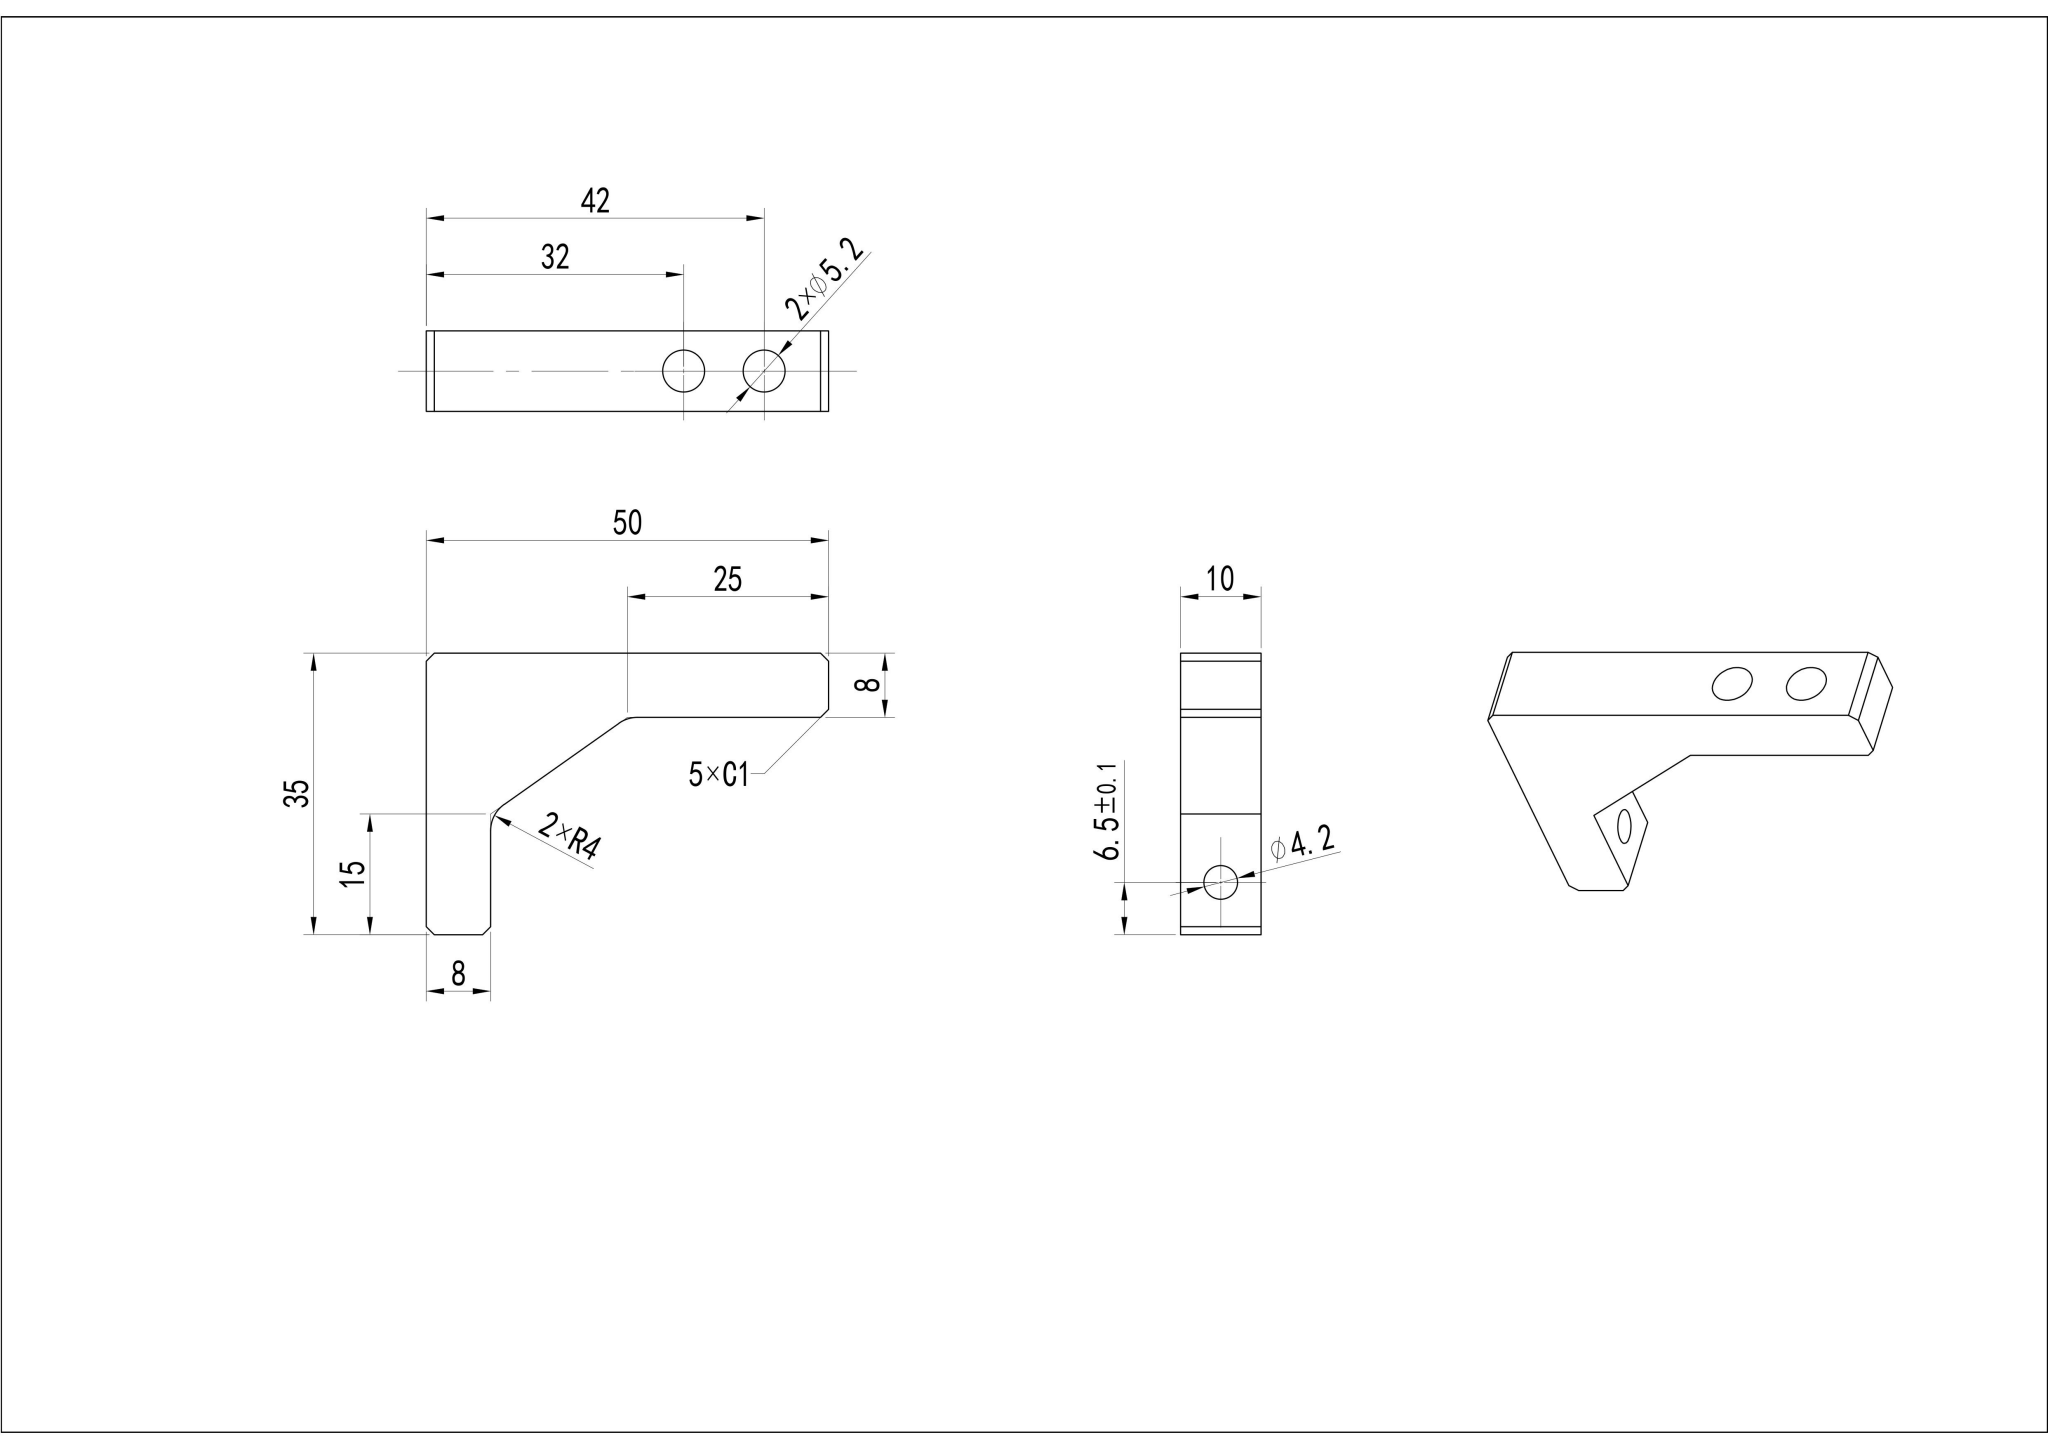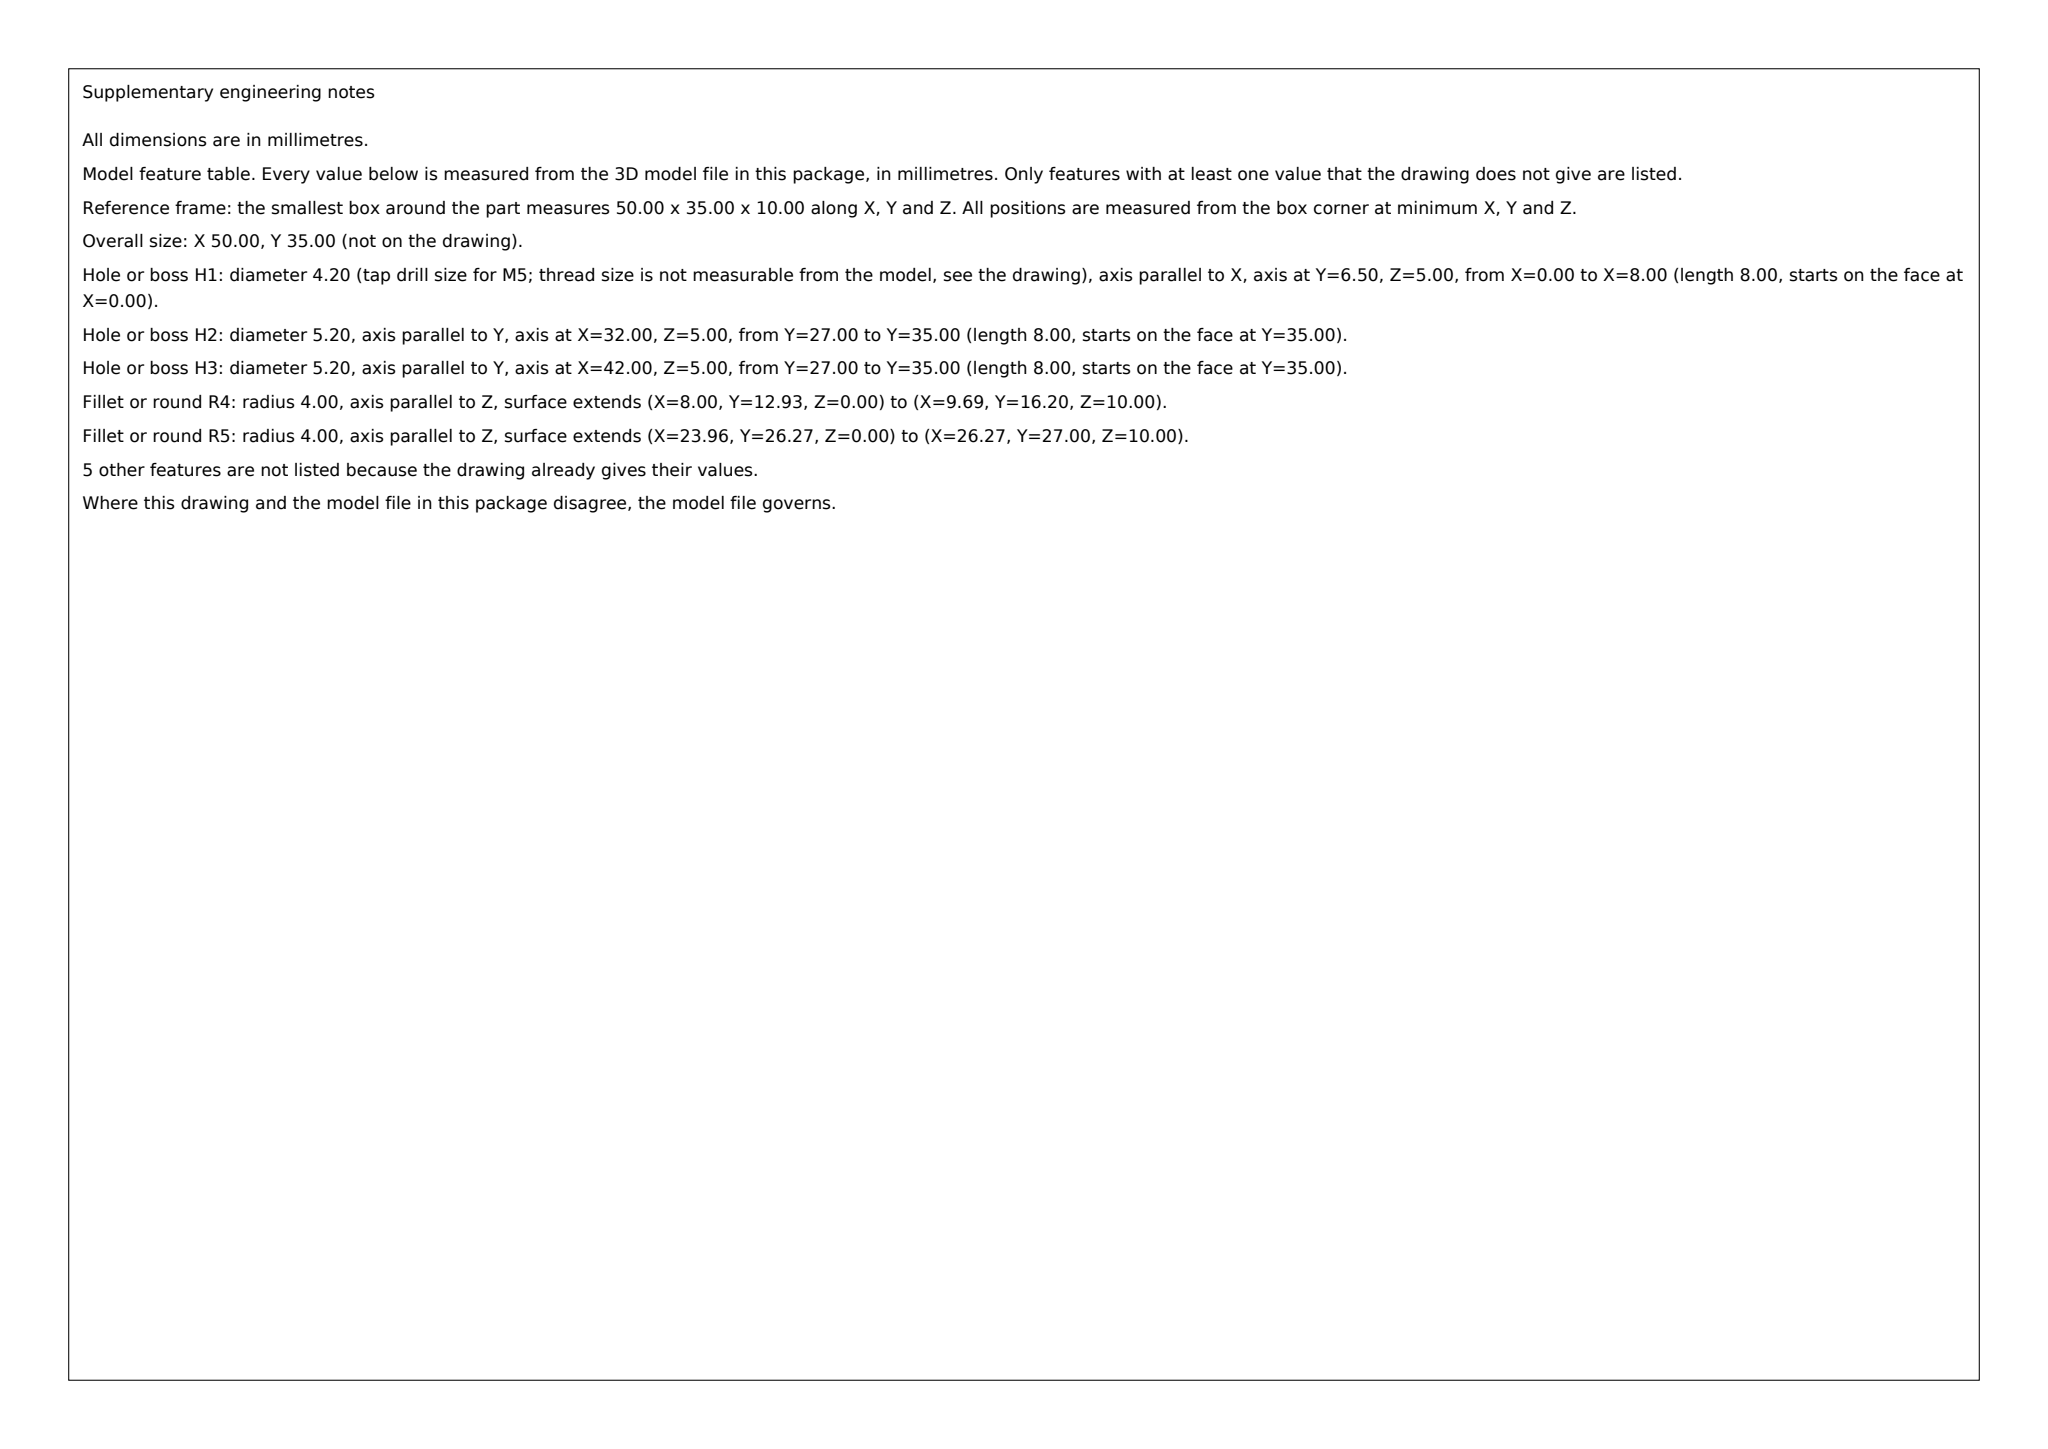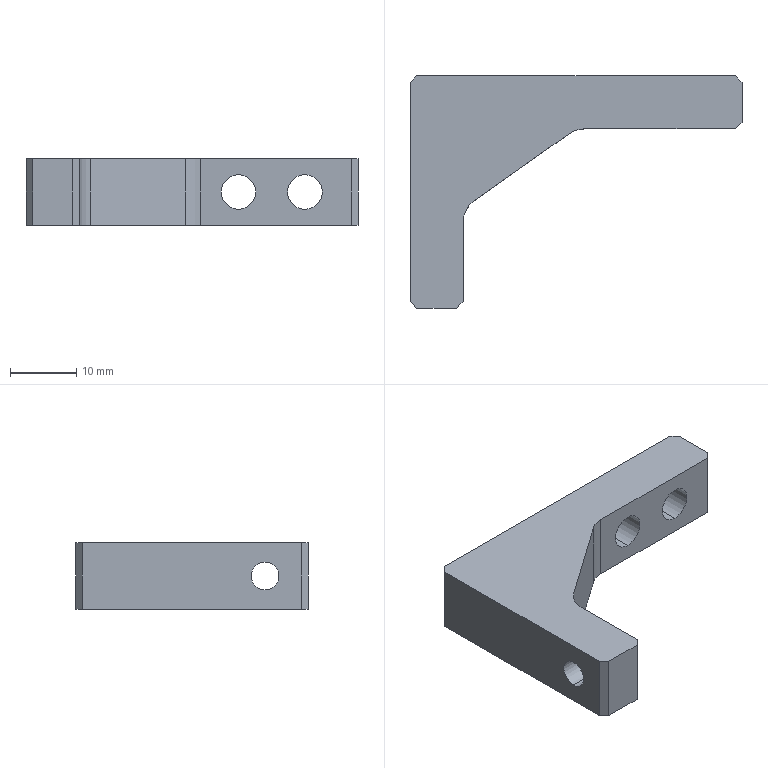Part | SolidWorks | mm | 1 solid | 22 faces | box 50 x 35 x 10 mm | volume 6712 mm3 | plane 14 | cylinder 8 | commonest cylinder face diameters 5.2 x4 4.2 x2 8 x2
STEP:
#1=CARTESIAN_POINT('',(-8.828,-14.732,2.1));
#2=VERTEX_POINT('',#1);
#3=CARTESIAN_POINT('',(-8.828,-14.732,-2.1));
#4=VERTEX_POINT('',#3);
#5=CARTESIAN_POINT('',(-8.828,-14.732,0.));
#6=DIRECTION('',(1.,0.,0.));
#7=DIRECTION('',(0.,0.,1.));
#8=AXIS2_PLACEMENT_3D('',#5,#6,#7);
#9=CIRCLE('',#8,2.1);
#10=EDGE_CURVE('',#2,#4,#9,.T.);
#11=ORIENTED_EDGE('',*,*,#10,.T.);
#12=CARTESIAN_POINT('',(-16.828,-14.732,-2.1));
#13=VERTEX_POINT('',#12);
#14=CARTESIAN_POINT('',(-6.828,-14.732,-2.1));
#15=DIRECTION('',(-1.,0.,0.));
#16=VECTOR('',#15,1000.);
#17=LINE('',#14,#16);
#18=EDGE_CURVE('',#4,#13,#17,.T.);
#19=ORIENTED_EDGE('',*,*,#18,.T.);
#20=CARTESIAN_POINT('',(-16.828,-14.732,2.1));
#21=VERTEX_POINT('',#20);
#22=CARTESIAN_POINT('',(-16.828,-14.732,0.));
#23=DIRECTION('',(-1.,0.,0.));
#24=DIRECTION('',(0.,0.,1.));
#25=AXIS2_PLACEMENT_3D('',#22,#23,#24);
#26=CIRCLE('',#25,2.1);
#27=EDGE_CURVE('',#13,#21,#26,.T.);
#28=ORIENTED_EDGE('',*,*,#27,.T.);
#29=CARTESIAN_POINT('',(-6.828,-14.732,2.1));
#30=DIRECTION('',(-1.,0.,0.));
#31=VECTOR('',#30,1000.);
#32=LINE('',#29,#31);
#33=EDGE_CURVE('',#2,#21,#32,.T.);
#34=ORIENTED_EDGE('',*,*,#33,.F.);
#35=EDGE_LOOP('',(#11,#19,#28,#34));
#36=FACE_OUTER_BOUND('',#35,.T.);
#37=CARTESIAN_POINT('',(-6.828,-14.732,0.));
#38=DIRECTION('',(-1.,0.,0.));
#39=DIRECTION('',(0.,0.,1.));
#40=AXIS2_PLACEMENT_3D('',#37,#38,#39);
#41=CYLINDRICAL_SURFACE('',#40,2.1);
#42=ADVANCED_FACE('',(#36),#41,.F.);
#43=CARTESIAN_POINT('',(15.172,5.768,2.6));
#44=VERTEX_POINT('',#43);
#45=CARTESIAN_POINT('',(15.172,5.768,-2.6));
#46=VERTEX_POINT('',#45);
#47=CARTESIAN_POINT('',(15.172,5.768,0.));
#48=DIRECTION('',(0.,-1.,0.));
#49=DIRECTION('',(0.,0.,1.));
#50=AXIS2_PLACEMENT_3D('',#47,#48,#49);
#51=CIRCLE('',#50,2.6);
#52=EDGE_CURVE('',#44,#46,#51,.T.);
#53=ORIENTED_EDGE('',*,*,#52,.T.);
#54=CARTESIAN_POINT('',(15.172,13.768,-2.6));
#55=VERTEX_POINT('',#54);
#56=CARTESIAN_POINT('',(15.172,3.768,-2.6));
#57=DIRECTION('',(0.,1.,0.));
#58=VECTOR('',#57,1000.);
#59=LINE('',#56,#58);
#60=EDGE_CURVE('',#46,#55,#59,.T.);
#61=ORIENTED_EDGE('',*,*,#60,.T.);
#62=CARTESIAN_POINT('',(15.172,13.768,2.6));
#63=VERTEX_POINT('',#62);
#64=CARTESIAN_POINT('',(15.172,13.768,0.));
#65=DIRECTION('',(0.,1.,0.));
#66=DIRECTION('',(0.,0.,1.));
#67=AXIS2_PLACEMENT_3D('',#64,#65,#66);
#68=CIRCLE('',#67,2.6);
#69=EDGE_CURVE('',#55,#63,#68,.T.);
#70=ORIENTED_EDGE('',*,*,#69,.T.);
#71=CARTESIAN_POINT('',(15.172,3.768,2.6));
#72=DIRECTION('',(0.,1.,0.));
#73=VECTOR('',#72,1000.);
#74=LINE('',#71,#73);
#75=EDGE_CURVE('',#44,#63,#74,.T.);
#76=ORIENTED_EDGE('',*,*,#75,.F.);
#77=EDGE_LOOP('',(#53,#61,#70,#76));
#78=FACE_OUTER_BOUND('',#77,.T.);
#79=CARTESIAN_POINT('',(15.172,3.768,0.));
#80=DIRECTION('',(0.,1.,0.));
#81=DIRECTION('',(0.,0.,1.));
#82=AXIS2_PLACEMENT_3D('',#79,#80,#81);
#83=CYLINDRICAL_SURFACE('',#82,2.6);
#84=ADVANCED_FACE('',(#78),#83,.F.);
#85=CARTESIAN_POINT('',(25.172,5.768,2.6));
#86=VERTEX_POINT('',#85);
#87=CARTESIAN_POINT('',(25.172,5.768,-2.6));
#88=VERTEX_POINT('',#87);
#89=CARTESIAN_POINT('',(25.172,5.768,0.));
#90=DIRECTION('',(0.,-1.,0.));
#91=DIRECTION('',(0.,0.,1.));
#92=AXIS2_PLACEMENT_3D('',#89,#90,#91);
#93=CIRCLE('',#92,2.6);
#94=EDGE_CURVE('',#86,#88,#93,.T.);
#95=ORIENTED_EDGE('',*,*,#94,.T.);
#96=CARTESIAN_POINT('',(25.172,13.768,-2.6));
#97=VERTEX_POINT('',#96);
#98=CARTESIAN_POINT('',(25.172,3.768,-2.6));
#99=DIRECTION('',(0.,1.,0.));
#100=VECTOR('',#99,1000.);
#101=LINE('',#98,#100);
#102=EDGE_CURVE('',#88,#97,#101,.T.);
#103=ORIENTED_EDGE('',*,*,#102,.T.);
#104=CARTESIAN_POINT('',(25.172,13.768,2.6));
#105=VERTEX_POINT('',#104);
#106=CARTESIAN_POINT('',(25.172,13.768,0.));
#107=DIRECTION('',(0.,1.,0.));
#108=DIRECTION('',(0.,0.,1.));
#109=AXIS2_PLACEMENT_3D('',#106,#107,#108);
#110=CIRCLE('',#109,2.6);
#111=EDGE_CURVE('',#97,#105,#110,.T.);
#112=ORIENTED_EDGE('',*,*,#111,.T.);
#113=CARTESIAN_POINT('',(25.172,3.768,2.6));
#114=DIRECTION('',(0.,1.,0.));
#115=VECTOR('',#114,1000.);
#116=LINE('',#113,#115);
#117=EDGE_CURVE('',#86,#105,#116,.T.);
#118=ORIENTED_EDGE('',*,*,#117,.F.);
#119=EDGE_LOOP('',(#95,#103,#112,#118));
#120=FACE_OUTER_BOUND('',#119,.T.);
#121=CARTESIAN_POINT('',(25.172,3.768,0.));
#122=DIRECTION('',(0.,1.,0.));
#123=DIRECTION('',(0.,0.,1.));
#124=AXIS2_PLACEMENT_3D('',#121,#122,#123);
#125=CYLINDRICAL_SURFACE('',#124,2.6);
#126=ADVANCED_FACE('',(#120),#125,.F.);
#127=CARTESIAN_POINT('',(-16.828,-20.232,5.));
#128=VERTEX_POINT('',#127);
#129=CARTESIAN_POINT('',(-15.828,-21.232,5.));
#130=VERTEX_POINT('',#129);
#131=CARTESIAN_POINT('',(-16.828,-20.232,5.));
#132=DIRECTION('',(0.7071,-0.7071,0.));
#133=VECTOR('',#132,1000.);
#134=LINE('',#131,#133);
#135=EDGE_CURVE('',#128,#130,#134,.T.);
#136=ORIENTED_EDGE('',*,*,#135,.T.);
#137=CARTESIAN_POINT('',(-9.828,-21.232,5.));
#138=VERTEX_POINT('',#137);
#139=CARTESIAN_POINT('',(-4.828,-21.232,5.));
#140=DIRECTION('',(-1.,0.,0.));
#141=VECTOR('',#140,1000.);
#142=LINE('',#139,#141);
#143=EDGE_CURVE('',#138,#130,#142,.T.);
#144=ORIENTED_EDGE('',*,*,#143,.F.);
#145=CARTESIAN_POINT('',(-8.828,-20.232,5.));
#146=VERTEX_POINT('',#145);
#147=CARTESIAN_POINT('',(-9.828,-21.232,5.));
#148=DIRECTION('',(0.7071,0.7071,0.));
#149=VECTOR('',#148,1000.);
#150=LINE('',#147,#149);
#151=EDGE_CURVE('',#138,#146,#150,.T.);
#152=ORIENTED_EDGE('',*,*,#151,.T.);
#153=CARTESIAN_POINT('',(-8.828,-8.304,5.));
#154=VERTEX_POINT('',#153);
#155=CARTESIAN_POINT('',(-8.828,-8.304,5.));
#156=DIRECTION('',(0.,-1.,0.));
#157=VECTOR('',#156,1000.);
#158=LINE('',#155,#157);
#159=EDGE_CURVE('',#154,#146,#158,.T.);
#160=ORIENTED_EDGE('',*,*,#159,.F.);
#161=CARTESIAN_POINT('',(-7.135,-5.036,5.));
#162=VERTEX_POINT('',#161);
#163=CARTESIAN_POINT('',(-4.828,-8.304,5.));
#164=DIRECTION('',(0.,0.,1.));
#165=DIRECTION('',(-1.,0.,0.));
#166=AXIS2_PLACEMENT_3D('',#163,#164,#165);
#167=CIRCLE('',#166,4.);
#168=EDGE_CURVE('',#162,#154,#167,.T.);
#169=ORIENTED_EDGE('',*,*,#168,.F.);
#170=CARTESIAN_POINT('',(7.135,5.036,5.));
#171=VERTEX_POINT('',#170);
#172=CARTESIAN_POINT('',(7.135,5.036,5.));
#173=DIRECTION('',(-0.817,-0.5767,0.));
#174=VECTOR('',#173,1000.);
#175=LINE('',#172,#174);
#176=EDGE_CURVE('',#171,#162,#175,.T.);
#177=ORIENTED_EDGE('',*,*,#176,.F.);
#178=CARTESIAN_POINT('',(9.442,5.768,5.));
#179=VERTEX_POINT('',#178);
#180=CARTESIAN_POINT('',(9.442,1.768,5.));
#181=DIRECTION('',(0.,0.,1.));
#182=DIRECTION('',(-1.,0.,0.));
#183=AXIS2_PLACEMENT_3D('',#180,#181,#182);
#184=CIRCLE('',#183,4.);
#185=EDGE_CURVE('',#179,#171,#184,.T.);
#186=ORIENTED_EDGE('',*,*,#185,.F.);
#187=CARTESIAN_POINT('',(32.172,5.768,5.));
#188=VERTEX_POINT('',#187);
#189=CARTESIAN_POINT('',(-4.828,5.768,5.));
#190=DIRECTION('',(-1.,0.,0.));
#191=VECTOR('',#190,1000.);
#192=LINE('',#189,#191);
#193=EDGE_CURVE('',#188,#179,#192,.T.);
#194=ORIENTED_EDGE('',*,*,#193,.F.);
#195=CARTESIAN_POINT('',(33.172,6.768,5.));
#196=VERTEX_POINT('',#195);
#197=CARTESIAN_POINT('',(32.172,5.768,5.));
#198=DIRECTION('',(0.7071,0.7071,0.));
#199=VECTOR('',#198,1000.);
#200=LINE('',#197,#199);
#201=EDGE_CURVE('',#188,#196,#200,.T.);
#202=ORIENTED_EDGE('',*,*,#201,.T.);
#203=CARTESIAN_POINT('',(33.172,12.768,5.));
#204=VERTEX_POINT('',#203);
#205=CARTESIAN_POINT('',(33.172,-8.304,5.));
#206=DIRECTION('',(0.,-1.,0.));
#207=VECTOR('',#206,1000.);
#208=LINE('',#205,#207);
#209=EDGE_CURVE('',#204,#196,#208,.T.);
#210=ORIENTED_EDGE('',*,*,#209,.F.);
#211=CARTESIAN_POINT('',(32.172,13.768,5.));
#212=VERTEX_POINT('',#211);
#213=CARTESIAN_POINT('',(33.172,12.768,5.));
#214=DIRECTION('',(-0.7071,0.7071,0.));
#215=VECTOR('',#214,1000.);
#216=LINE('',#213,#215);
#217=EDGE_CURVE('',#204,#212,#216,.T.);
#218=ORIENTED_EDGE('',*,*,#217,.T.);
#219=CARTESIAN_POINT('',(-15.828,13.768,5.));
#220=VERTEX_POINT('',#219);
#221=CARTESIAN_POINT('',(-4.828,13.768,5.));
#222=DIRECTION('',(1.,0.,0.));
#223=VECTOR('',#222,1000.);
#224=LINE('',#221,#223);
#225=EDGE_CURVE('',#220,#212,#224,.T.);
#226=ORIENTED_EDGE('',*,*,#225,.F.);
#227=CARTESIAN_POINT('',(-16.828,12.768,5.));
#228=VERTEX_POINT('',#227);
#229=CARTESIAN_POINT('',(-15.828,13.768,5.));
#230=DIRECTION('',(-0.7071,-0.7071,0.));
#231=VECTOR('',#230,1000.);
#232=LINE('',#229,#231);
#233=EDGE_CURVE('',#220,#228,#232,.T.);
#234=ORIENTED_EDGE('',*,*,#233,.T.);
#235=CARTESIAN_POINT('',(-16.828,-8.304,5.));
#236=DIRECTION('',(0.,1.,0.));
#237=VECTOR('',#236,1000.);
#238=LINE('',#235,#237);
#239=EDGE_CURVE('',#128,#228,#238,.T.);
#240=ORIENTED_EDGE('',*,*,#239,.F.);
#241=EDGE_LOOP('',(#136,#144,#152,#160,#169,#177,#186,#194,#202,#210,#218,#226,#234,#240));
#242=FACE_OUTER_BOUND('',#241,.T.);
#243=CARTESIAN_POINT('',(-4.828,-8.304,5.));
#244=DIRECTION('',(0.,0.,-1.));
#245=DIRECTION('',(-1.,0.,0.));
#246=AXIS2_PLACEMENT_3D('',#243,#244,#245);
#247=PLANE('',#246);
#248=ADVANCED_FACE('',(#242),#247,.F.);
#249=CARTESIAN_POINT('',(-16.828,-20.232,-5.));
#250=VERTEX_POINT('',#249);
#251=CARTESIAN_POINT('',(-16.828,-20.232,5.));
#252=DIRECTION('',(0.,0.,-1.));
#253=VECTOR('',#252,1000.);
#254=LINE('',#251,#253);
#255=EDGE_CURVE('',#128,#250,#254,.T.);
#256=ORIENTED_EDGE('',*,*,#255,.F.);
#257=ORIENTED_EDGE('',*,*,#239,.T.);
#258=CARTESIAN_POINT('',(-16.828,12.768,-5.));
#259=VERTEX_POINT('',#258);
#260=CARTESIAN_POINT('',(-16.828,12.768,5.));
#261=DIRECTION('',(0.,0.,1.));
#262=VECTOR('',#261,1000.);
#263=LINE('',#260,#262);
#264=EDGE_CURVE('',#259,#228,#263,.T.);
#265=ORIENTED_EDGE('',*,*,#264,.F.);
#266=CARTESIAN_POINT('',(-16.828,12.768,-5.));
#267=DIRECTION('',(0.,1.,0.));
#268=VECTOR('',#267,1000.);
#269=LINE('',#266,#268);
#270=EDGE_CURVE('',#250,#259,#269,.T.);
#271=ORIENTED_EDGE('',*,*,#270,.F.);
#272=EDGE_LOOP('',(#256,#257,#265,#271));
#273=FACE_OUTER_BOUND('',#272,.T.);
#274=CARTESIAN_POINT('',(-16.828,-14.732,0.));
#275=DIRECTION('',(-1.,0.,0.));
#276=DIRECTION('',(0.,0.,1.));
#277=AXIS2_PLACEMENT_3D('',#274,#275,#276);
#278=CIRCLE('',#277,2.1);
#279=EDGE_CURVE('',#21,#13,#278,.T.);
#280=ORIENTED_EDGE('',*,*,#279,.F.);
#281=ORIENTED_EDGE('',*,*,#27,.F.);
#282=EDGE_LOOP('',(#280,#281));
#283=FACE_BOUND('',#282,.T.);
#284=CARTESIAN_POINT('',(-16.828,12.768,5.));
#285=DIRECTION('',(1.,0.,0.));
#286=DIRECTION('',(0.,0.,-1.));
#287=AXIS2_PLACEMENT_3D('',#284,#285,#286);
#288=PLANE('',#287);
#289=ADVANCED_FACE('',(#273,#283),#288,.F.);
#290=CARTESIAN_POINT('',(-9.828,-21.232,-5.));
#291=VERTEX_POINT('',#290);
#292=CARTESIAN_POINT('',(-9.828,-21.232,5.));
#293=DIRECTION('',(0.,0.,-1.));
#294=VECTOR('',#293,1000.);
#295=LINE('',#292,#294);
#296=EDGE_CURVE('',#138,#291,#295,.T.);
#297=ORIENTED_EDGE('',*,*,#296,.F.);
#298=ORIENTED_EDGE('',*,*,#143,.T.);
#299=CARTESIAN_POINT('',(-15.828,-21.232,-5.));
#300=VERTEX_POINT('',#299);
#301=CARTESIAN_POINT('',(-15.828,-21.232,5.));
#302=DIRECTION('',(0.,0.,1.));
#303=VECTOR('',#302,1000.);
#304=LINE('',#301,#303);
#305=EDGE_CURVE('',#300,#130,#304,.T.);
#306=ORIENTED_EDGE('',*,*,#305,.F.);
#307=CARTESIAN_POINT('',(-15.828,-21.232,-5.));
#308=DIRECTION('',(-1.,0.,0.));
#309=VECTOR('',#308,1000.);
#310=LINE('',#307,#309);
#311=EDGE_CURVE('',#291,#300,#310,.T.);
#312=ORIENTED_EDGE('',*,*,#311,.F.);
#313=EDGE_LOOP('',(#297,#298,#306,#312));
#314=FACE_OUTER_BOUND('',#313,.T.);
#315=CARTESIAN_POINT('',(-15.828,-21.232,5.));
#316=DIRECTION('',(0.,1.,0.));
#317=DIRECTION('',(0.,0.,1.));
#318=AXIS2_PLACEMENT_3D('',#315,#316,#317);
#319=PLANE('',#318);
#320=ADVANCED_FACE('',(#314),#319,.F.);
#321=CARTESIAN_POINT('',(-8.828,-8.304,-5.));
#322=VERTEX_POINT('',#321);
#323=CARTESIAN_POINT('',(-8.828,-8.304,5.));
#324=DIRECTION('',(0.,0.,-1.));
#325=VECTOR('',#324,1000.);
#326=LINE('',#323,#325);
#327=EDGE_CURVE('',#154,#322,#326,.T.);
#328=ORIENTED_EDGE('',*,*,#327,.F.);
#329=ORIENTED_EDGE('',*,*,#159,.T.);
#330=CARTESIAN_POINT('',(-8.828,-20.232,-5.));
#331=VERTEX_POINT('',#330);
#332=CARTESIAN_POINT('',(-8.828,-20.232,5.));
#333=DIRECTION('',(0.,0.,1.));
#334=VECTOR('',#333,1000.);
#335=LINE('',#332,#334);
#336=EDGE_CURVE('',#331,#146,#335,.T.);
#337=ORIENTED_EDGE('',*,*,#336,.F.);
#338=CARTESIAN_POINT('',(-8.828,-20.232,-5.));
#339=DIRECTION('',(0.,-1.,0.));
#340=VECTOR('',#339,1000.);
#341=LINE('',#338,#340);
#342=EDGE_CURVE('',#322,#331,#341,.T.);
#343=ORIENTED_EDGE('',*,*,#342,.F.);
#344=EDGE_LOOP('',(#328,#329,#337,#343));
#345=FACE_OUTER_BOUND('',#344,.T.);
#346=ORIENTED_EDGE('',*,*,#10,.F.);
#347=CARTESIAN_POINT('',(-8.828,-14.732,0.));
#348=DIRECTION('',(1.,0.,0.));
#349=DIRECTION('',(0.,0.,1.));
#350=AXIS2_PLACEMENT_3D('',#347,#348,#349);
#351=CIRCLE('',#350,2.1);
#352=EDGE_CURVE('',#4,#2,#351,.T.);
#353=ORIENTED_EDGE('',*,*,#352,.F.);
#354=EDGE_LOOP('',(#346,#353));
#355=FACE_BOUND('',#354,.T.);
#356=CARTESIAN_POINT('',(-8.828,-20.232,5.));
#357=DIRECTION('',(-1.,-0.,0.));
#358=DIRECTION('',(0.,-1.,0.));
#359=AXIS2_PLACEMENT_3D('',#356,#357,#358);
#360=PLANE('',#359);
#361=ADVANCED_FACE('',(#345,#355),#360,.F.);
#362=CARTESIAN_POINT('',(-7.135,-5.036,-5.));
#363=VERTEX_POINT('',#362);
#364=CARTESIAN_POINT('',(-7.135,-5.036,5.));
#365=DIRECTION('',(0.,0.,-1.));
#366=VECTOR('',#365,1000.);
#367=LINE('',#364,#366);
#368=EDGE_CURVE('',#162,#363,#367,.T.);
#369=ORIENTED_EDGE('',*,*,#368,.F.);
#370=ORIENTED_EDGE('',*,*,#168,.T.);
#371=ORIENTED_EDGE('',*,*,#327,.T.);
#372=CARTESIAN_POINT('',(-4.828,-8.304,-5.));
#373=DIRECTION('',(0.,0.,1.));
#374=DIRECTION('',(-1.,0.,0.));
#375=AXIS2_PLACEMENT_3D('',#372,#373,#374);
#376=CIRCLE('',#375,4.);
#377=EDGE_CURVE('',#363,#322,#376,.T.);
#378=ORIENTED_EDGE('',*,*,#377,.F.);
#379=EDGE_LOOP('',(#369,#370,#371,#378));
#380=FACE_OUTER_BOUND('',#379,.T.);
#381=CARTESIAN_POINT('',(-4.828,-8.304,5.));
#382=DIRECTION('',(0.,0.,-1.));
#383=DIRECTION('',(-1.,0.,0.));
#384=AXIS2_PLACEMENT_3D('',#381,#382,#383);
#385=CYLINDRICAL_SURFACE('',#384,4.);
#386=ADVANCED_FACE('',(#380),#385,.F.);
#387=CARTESIAN_POINT('',(7.135,5.036,-5.));
#388=VERTEX_POINT('',#387);
#389=CARTESIAN_POINT('',(7.135,5.036,5.));
#390=DIRECTION('',(0.,0.,-1.));
#391=VECTOR('',#390,1000.);
#392=LINE('',#389,#391);
#393=EDGE_CURVE('',#171,#388,#392,.T.);
#394=ORIENTED_EDGE('',*,*,#393,.F.);
#395=ORIENTED_EDGE('',*,*,#176,.T.);
#396=ORIENTED_EDGE('',*,*,#368,.T.);
#397=CARTESIAN_POINT('',(-7.135,-5.036,-5.));
#398=DIRECTION('',(-0.817,-0.5767,0.));
#399=VECTOR('',#398,1000.);
#400=LINE('',#397,#399);
#401=EDGE_CURVE('',#388,#363,#400,.T.);
#402=ORIENTED_EDGE('',*,*,#401,.F.);
#403=EDGE_LOOP('',(#394,#395,#396,#402));
#404=FACE_OUTER_BOUND('',#403,.T.);
#405=CARTESIAN_POINT('',(-7.135,-5.036,5.));
#406=DIRECTION('',(-0.5767,0.817,0.));
#407=DIRECTION('',(-0.817,-0.5767,0.));
#408=AXIS2_PLACEMENT_3D('',#405,#406,#407);
#409=PLANE('',#408);
#410=ADVANCED_FACE('',(#404),#409,.F.);
#411=CARTESIAN_POINT('',(9.442,5.768,-5.));
#412=VERTEX_POINT('',#411);
#413=CARTESIAN_POINT('',(9.442,5.768,5.));
#414=DIRECTION('',(0.,0.,-1.));
#415=VECTOR('',#414,1000.);
#416=LINE('',#413,#415);
#417=EDGE_CURVE('',#179,#412,#416,.T.);
#418=ORIENTED_EDGE('',*,*,#417,.F.);
#419=ORIENTED_EDGE('',*,*,#185,.T.);
#420=ORIENTED_EDGE('',*,*,#393,.T.);
#421=CARTESIAN_POINT('',(9.442,1.768,-5.));
#422=DIRECTION('',(0.,0.,1.));
#423=DIRECTION('',(-1.,-0.,0.));
#424=AXIS2_PLACEMENT_3D('',#421,#422,#423);
#425=CIRCLE('',#424,4.);
#426=EDGE_CURVE('',#412,#388,#425,.T.);
#427=ORIENTED_EDGE('',*,*,#426,.F.);
#428=EDGE_LOOP('',(#418,#419,#420,#427));
#429=FACE_OUTER_BOUND('',#428,.T.);
#430=CARTESIAN_POINT('',(9.442,1.768,5.));
#431=DIRECTION('',(0.,0.,-1.));
#432=DIRECTION('',(-1.,0.,0.));
#433=AXIS2_PLACEMENT_3D('',#430,#431,#432);
#434=CYLINDRICAL_SURFACE('',#433,4.);
#435=ADVANCED_FACE('',(#429),#434,.F.);
#436=CARTESIAN_POINT('',(32.172,5.768,-5.));
#437=VERTEX_POINT('',#436);
#438=CARTESIAN_POINT('',(32.172,5.768,5.));
#439=DIRECTION('',(0.,0.,-1.));
#440=VECTOR('',#439,1000.);
#441=LINE('',#438,#440);
#442=EDGE_CURVE('',#188,#437,#441,.T.);
#443=ORIENTED_EDGE('',*,*,#442,.F.);
#444=ORIENTED_EDGE('',*,*,#193,.T.);
#445=ORIENTED_EDGE('',*,*,#417,.T.);
#446=CARTESIAN_POINT('',(9.442,5.768,-5.));
#447=DIRECTION('',(-1.,0.,0.));
#448=VECTOR('',#447,1000.);
#449=LINE('',#446,#448);
#450=EDGE_CURVE('',#437,#412,#449,.T.);
#451=ORIENTED_EDGE('',*,*,#450,.F.);
#452=EDGE_LOOP('',(#443,#444,#445,#451));
#453=FACE_OUTER_BOUND('',#452,.T.);
#454=ORIENTED_EDGE('',*,*,#52,.F.);
#455=CARTESIAN_POINT('',(15.172,5.768,0.));
#456=DIRECTION('',(0.,-1.,0.));
#457=DIRECTION('',(0.,0.,1.));
#458=AXIS2_PLACEMENT_3D('',#455,#456,#457);
#459=CIRCLE('',#458,2.6);
#460=EDGE_CURVE('',#46,#44,#459,.T.);
#461=ORIENTED_EDGE('',*,*,#460,.F.);
#462=EDGE_LOOP('',(#454,#461));
#463=FACE_BOUND('',#462,.T.);
#464=ORIENTED_EDGE('',*,*,#94,.F.);
#465=CARTESIAN_POINT('',(25.172,5.768,0.));
#466=DIRECTION('',(0.,-1.,0.));
#467=DIRECTION('',(0.,0.,1.));
#468=AXIS2_PLACEMENT_3D('',#465,#466,#467);
#469=CIRCLE('',#468,2.6);
#470=EDGE_CURVE('',#88,#86,#469,.T.);
#471=ORIENTED_EDGE('',*,*,#470,.F.);
#472=EDGE_LOOP('',(#464,#471));
#473=FACE_BOUND('',#472,.T.);
#474=CARTESIAN_POINT('',(9.442,5.768,5.));
#475=DIRECTION('',(0.,1.,0.));
#476=DIRECTION('',(0.,0.,1.));
#477=AXIS2_PLACEMENT_3D('',#474,#475,#476);
#478=PLANE('',#477);
#479=ADVANCED_FACE('',(#453,#463,#473),#478,.F.);
#480=CARTESIAN_POINT('',(33.172,12.768,-5.));
#481=VERTEX_POINT('',#480);
#482=CARTESIAN_POINT('',(33.172,12.768,5.));
#483=DIRECTION('',(0.,0.,-1.));
#484=VECTOR('',#483,1000.);
#485=LINE('',#482,#484);
#486=EDGE_CURVE('',#204,#481,#485,.T.);
#487=ORIENTED_EDGE('',*,*,#486,.F.);
#488=ORIENTED_EDGE('',*,*,#209,.T.);
#489=CARTESIAN_POINT('',(33.172,6.768,-5.));
#490=VERTEX_POINT('',#489);
#491=CARTESIAN_POINT('',(33.172,6.768,5.));
#492=DIRECTION('',(0.,0.,1.));
#493=VECTOR('',#492,1000.);
#494=LINE('',#491,#493);
#495=EDGE_CURVE('',#490,#196,#494,.T.);
#496=ORIENTED_EDGE('',*,*,#495,.F.);
#497=CARTESIAN_POINT('',(33.172,6.768,-5.));
#498=DIRECTION('',(0.,-1.,0.));
#499=VECTOR('',#498,1000.);
#500=LINE('',#497,#499);
#501=EDGE_CURVE('',#481,#490,#500,.T.);
#502=ORIENTED_EDGE('',*,*,#501,.F.);
#503=EDGE_LOOP('',(#487,#488,#496,#502));
#504=FACE_OUTER_BOUND('',#503,.T.);
#505=CARTESIAN_POINT('',(33.172,6.768,5.));
#506=DIRECTION('',(-1.,0.,0.));
#507=DIRECTION('',(0.,0.,1.));
#508=AXIS2_PLACEMENT_3D('',#505,#506,#507);
#509=PLANE('',#508);
#510=ADVANCED_FACE('',(#504),#509,.F.);
#511=CARTESIAN_POINT('',(-15.828,13.768,-5.));
#512=VERTEX_POINT('',#511);
#513=CARTESIAN_POINT('',(-15.828,13.768,5.));
#514=DIRECTION('',(0.,0.,-1.));
#515=VECTOR('',#514,1000.);
#516=LINE('',#513,#515);
#517=EDGE_CURVE('',#220,#512,#516,.T.);
#518=ORIENTED_EDGE('',*,*,#517,.F.);
#519=ORIENTED_EDGE('',*,*,#225,.T.);
#520=CARTESIAN_POINT('',(32.172,13.768,-5.));
#521=VERTEX_POINT('',#520);
#522=CARTESIAN_POINT('',(32.172,13.768,5.));
#523=DIRECTION('',(0.,0.,1.));
#524=VECTOR('',#523,1000.);
#525=LINE('',#522,#524);
#526=EDGE_CURVE('',#521,#212,#525,.T.);
#527=ORIENTED_EDGE('',*,*,#526,.F.);
#528=CARTESIAN_POINT('',(32.172,13.768,-5.));
#529=DIRECTION('',(1.,0.,0.));
#530=VECTOR('',#529,1000.);
#531=LINE('',#528,#530);
#532=EDGE_CURVE('',#512,#521,#531,.T.);
#533=ORIENTED_EDGE('',*,*,#532,.F.);
#534=EDGE_LOOP('',(#518,#519,#527,#533));
#535=FACE_OUTER_BOUND('',#534,.T.);
#536=CARTESIAN_POINT('',(15.172,13.768,0.));
#537=DIRECTION('',(0.,1.,0.));
#538=DIRECTION('',(0.,0.,1.));
#539=AXIS2_PLACEMENT_3D('',#536,#537,#538);
#540=CIRCLE('',#539,2.6);
#541=EDGE_CURVE('',#63,#55,#540,.T.);
#542=ORIENTED_EDGE('',*,*,#541,.F.);
#543=ORIENTED_EDGE('',*,*,#69,.F.);
#544=EDGE_LOOP('',(#542,#543));
#545=FACE_BOUND('',#544,.T.);
#546=CARTESIAN_POINT('',(25.172,13.768,0.));
#547=DIRECTION('',(0.,1.,0.));
#548=DIRECTION('',(0.,0.,1.));
#549=AXIS2_PLACEMENT_3D('',#546,#547,#548);
#550=CIRCLE('',#549,2.6);
#551=EDGE_CURVE('',#105,#97,#550,.T.);
#552=ORIENTED_EDGE('',*,*,#551,.F.);
#553=ORIENTED_EDGE('',*,*,#111,.F.);
#554=EDGE_LOOP('',(#552,#553));
#555=FACE_BOUND('',#554,.T.);
#556=CARTESIAN_POINT('',(32.172,13.768,5.));
#557=DIRECTION('',(0.,-1.,0.));
#558=DIRECTION('',(0.,0.,-1.));
#559=AXIS2_PLACEMENT_3D('',#556,#557,#558);
#560=PLANE('',#559);
#561=ADVANCED_FACE('',(#535,#545,#555),#560,.F.);
#562=ORIENTED_EDGE('',*,*,#311,.T.);
#563=CARTESIAN_POINT('',(-15.828,-21.232,-5.));
#564=DIRECTION('',(-0.7071,0.7071,0.));
#565=VECTOR('',#564,1000.);
#566=LINE('',#563,#565);
#567=EDGE_CURVE('',#300,#250,#566,.T.);
#568=ORIENTED_EDGE('',*,*,#567,.T.);
#569=ORIENTED_EDGE('',*,*,#270,.T.);
#570=CARTESIAN_POINT('',(-16.828,12.768,-5.));
#571=DIRECTION('',(0.7071,0.7071,0.));
#572=VECTOR('',#571,1000.);
#573=LINE('',#570,#572);
#574=EDGE_CURVE('',#259,#512,#573,.T.);
#575=ORIENTED_EDGE('',*,*,#574,.T.);
#576=ORIENTED_EDGE('',*,*,#532,.T.);
#577=CARTESIAN_POINT('',(32.172,13.768,-5.));
#578=DIRECTION('',(0.7071,-0.7071,0.));
#579=VECTOR('',#578,1000.);
#580=LINE('',#577,#579);
#581=EDGE_CURVE('',#521,#481,#580,.T.);
#582=ORIENTED_EDGE('',*,*,#581,.T.);
#583=ORIENTED_EDGE('',*,*,#501,.T.);
#584=CARTESIAN_POINT('',(33.172,6.768,-5.));
#585=DIRECTION('',(-0.7071,-0.7071,0.));
#586=VECTOR('',#585,1000.);
#587=LINE('',#584,#586);
#588=EDGE_CURVE('',#490,#437,#587,.T.);
#589=ORIENTED_EDGE('',*,*,#588,.T.);
#590=ORIENTED_EDGE('',*,*,#450,.T.);
#591=ORIENTED_EDGE('',*,*,#426,.T.);
#592=ORIENTED_EDGE('',*,*,#401,.T.);
#593=ORIENTED_EDGE('',*,*,#377,.T.);
#594=ORIENTED_EDGE('',*,*,#342,.T.);
#595=CARTESIAN_POINT('',(-8.828,-20.232,-5.));
#596=DIRECTION('',(-0.7071,-0.7071,0.));
#597=VECTOR('',#596,1000.);
#598=LINE('',#595,#597);
#599=EDGE_CURVE('',#331,#291,#598,.T.);
#600=ORIENTED_EDGE('',*,*,#599,.T.);
#601=EDGE_LOOP('',(#562,#568,#569,#575,#576,#582,#583,#589,#590,#591,#592,#593,#594,#600));
#602=FACE_OUTER_BOUND('',#601,.T.);
#603=CARTESIAN_POINT('',(-4.828,-8.304,-5.));
#604=DIRECTION('',(0.,0.,-1.));
#605=DIRECTION('',(-1.,0.,0.));
#606=AXIS2_PLACEMENT_3D('',#603,#604,#605);
#607=PLANE('',#606);
#608=ADVANCED_FACE('',(#602),#607,.T.);
#609=ORIENTED_EDGE('',*,*,#305,.T.);
#610=ORIENTED_EDGE('',*,*,#135,.F.);
#611=ORIENTED_EDGE('',*,*,#255,.T.);
#612=ORIENTED_EDGE('',*,*,#567,.F.);
#613=EDGE_LOOP('',(#609,#610,#611,#612));
#614=FACE_OUTER_BOUND('',#613,.T.);
#615=CARTESIAN_POINT('',(-16.828,-20.232,5.));
#616=DIRECTION('',(0.7071,0.7071,0.));
#617=DIRECTION('',(-0.7071,0.7071,0.));
#618=AXIS2_PLACEMENT_3D('',#615,#616,#617);
#619=PLANE('',#618);
#620=ADVANCED_FACE('',(#614),#619,.F.);
#621=ORIENTED_EDGE('',*,*,#264,.T.);
#622=ORIENTED_EDGE('',*,*,#233,.F.);
#623=ORIENTED_EDGE('',*,*,#517,.T.);
#624=ORIENTED_EDGE('',*,*,#574,.F.);
#625=EDGE_LOOP('',(#621,#622,#623,#624));
#626=FACE_OUTER_BOUND('',#625,.T.);
#627=CARTESIAN_POINT('',(-15.828,13.768,5.));
#628=DIRECTION('',(0.7071,-0.7071,0.));
#629=DIRECTION('',(0.7071,0.7071,0.));
#630=AXIS2_PLACEMENT_3D('',#627,#628,#629);
#631=PLANE('',#630);
#632=ADVANCED_FACE('',(#626),#631,.F.);
#633=ORIENTED_EDGE('',*,*,#18,.F.);
#634=ORIENTED_EDGE('',*,*,#352,.T.);
#635=ORIENTED_EDGE('',*,*,#33,.T.);
#636=ORIENTED_EDGE('',*,*,#279,.T.);
#637=EDGE_LOOP('',(#633,#634,#635,#636));
#638=FACE_OUTER_BOUND('',#637,.T.);
#639=CARTESIAN_POINT('',(-6.828,-14.732,0.));
#640=DIRECTION('',(-1.,0.,0.));
#641=DIRECTION('',(0.,0.,1.));
#642=AXIS2_PLACEMENT_3D('',#639,#640,#641);
#643=CYLINDRICAL_SURFACE('',#642,2.1);
#644=ADVANCED_FACE('',(#638),#643,.F.);
#645=ORIENTED_EDGE('',*,*,#336,.T.);
#646=ORIENTED_EDGE('',*,*,#151,.F.);
#647=ORIENTED_EDGE('',*,*,#296,.T.);
#648=ORIENTED_EDGE('',*,*,#599,.F.);
#649=EDGE_LOOP('',(#645,#646,#647,#648));
#650=FACE_OUTER_BOUND('',#649,.T.);
#651=CARTESIAN_POINT('',(-9.828,-21.232,5.));
#652=DIRECTION('',(-0.7071,0.7071,0.));
#653=DIRECTION('',(-0.7071,-0.7071,0.));
#654=AXIS2_PLACEMENT_3D('',#651,#652,#653);
#655=PLANE('',#654);
#656=ADVANCED_FACE('',(#650),#655,.F.);
#657=ORIENTED_EDGE('',*,*,#495,.T.);
#658=ORIENTED_EDGE('',*,*,#201,.F.);
#659=ORIENTED_EDGE('',*,*,#442,.T.);
#660=ORIENTED_EDGE('',*,*,#588,.F.);
#661=EDGE_LOOP('',(#657,#658,#659,#660));
#662=FACE_OUTER_BOUND('',#661,.T.);
#663=CARTESIAN_POINT('',(32.172,5.768,5.));
#664=DIRECTION('',(-0.7071,0.7071,0.));
#665=DIRECTION('',(-0.7071,-0.7071,0.));
#666=AXIS2_PLACEMENT_3D('',#663,#664,#665);
#667=PLANE('',#666);
#668=ADVANCED_FACE('',(#662),#667,.F.);
#669=ORIENTED_EDGE('',*,*,#60,.F.);
#670=ORIENTED_EDGE('',*,*,#460,.T.);
#671=ORIENTED_EDGE('',*,*,#75,.T.);
#672=ORIENTED_EDGE('',*,*,#541,.T.);
#673=EDGE_LOOP('',(#669,#670,#671,#672));
#674=FACE_OUTER_BOUND('',#673,.T.);
#675=CARTESIAN_POINT('',(15.172,3.768,0.));
#676=DIRECTION('',(0.,1.,0.));
#677=DIRECTION('',(0.,0.,1.));
#678=AXIS2_PLACEMENT_3D('',#675,#676,#677);
#679=CYLINDRICAL_SURFACE('',#678,2.6);
#680=ADVANCED_FACE('',(#674),#679,.F.);
#681=ORIENTED_EDGE('',*,*,#102,.F.);
#682=ORIENTED_EDGE('',*,*,#470,.T.);
#683=ORIENTED_EDGE('',*,*,#117,.T.);
#684=ORIENTED_EDGE('',*,*,#551,.T.);
#685=EDGE_LOOP('',(#681,#682,#683,#684));
#686=FACE_OUTER_BOUND('',#685,.T.);
#687=CARTESIAN_POINT('',(25.172,3.768,0.));
#688=DIRECTION('',(0.,1.,0.));
#689=DIRECTION('',(0.,0.,1.));
#690=AXIS2_PLACEMENT_3D('',#687,#688,#689);
#691=CYLINDRICAL_SURFACE('',#690,2.6);
#692=ADVANCED_FACE('',(#686),#691,.F.);
#693=ORIENTED_EDGE('',*,*,#526,.T.);
#694=ORIENTED_EDGE('',*,*,#217,.F.);
#695=ORIENTED_EDGE('',*,*,#486,.T.);
#696=ORIENTED_EDGE('',*,*,#581,.F.);
#697=EDGE_LOOP('',(#693,#694,#695,#696));
#698=FACE_OUTER_BOUND('',#697,.T.);
#699=CARTESIAN_POINT('',(33.172,12.768,5.));
#700=DIRECTION('',(-0.7071,-0.7071,0.));
#701=DIRECTION('',(0.7071,-0.7071,0.));
#702=AXIS2_PLACEMENT_3D('',#699,#700,#701);
#703=PLANE('',#702);
#704=ADVANCED_FACE('',(#698),#703,.F.);
#705=CLOSED_SHELL('',(#42,#84,#126,#248,#289,#320,#361,#386,#410,#435,#479,#510,#561,#608,#620,#632,#644,#656,#668,#680,#692,#704));
#706=MANIFOLD_SOLID_BREP('',#705);
#707=CARTESIAN_POINT('',(0.,0.,0.));
#708=DIRECTION('',(0.,0.,1.));
#709=DIRECTION('',(1.,0.,0.));
#710=AXIS2_PLACEMENT_3D('',#707,#708,#709);
#711=(LENGTH_UNIT()NAMED_UNIT(*)SI_UNIT(.MILLI.,.METRE.));
#712=UNCERTAINTY_MEASURE_WITH_UNIT(LENGTH_MEASURE(0.00001),#711,'','');
#713=(NAMED_UNIT(*)PLANE_ANGLE_UNIT()SI_UNIT($,.RADIAN.));
#714=(NAMED_UNIT(*)SI_UNIT($,.STERADIAN.)SOLID_ANGLE_UNIT());
#715=(GEOMETRIC_REPRESENTATION_CONTEXT(3)GLOBAL_UNCERTAINTY_ASSIGNED_CONTEXT((#712))GLOBAL_UNIT_ASSIGNED_CONTEXT((#711,#713,#714))REPRESENTATION_CONTEXT('',''));
#716=ADVANCED_BREP_SHAPE_REPRESENTATION('',(#706,#710),#715);